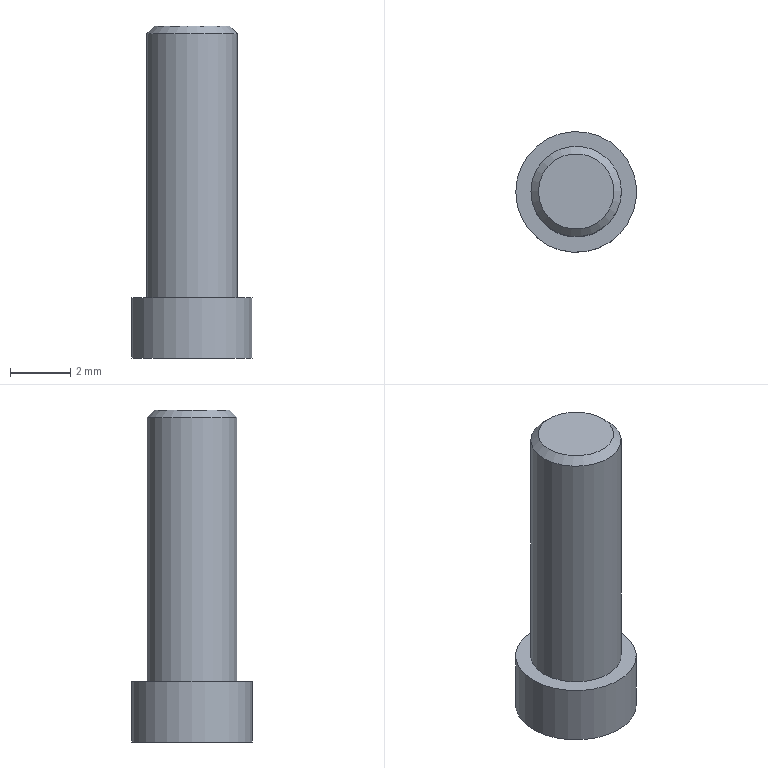Component | NX | SCREW_M3X7_11 | 1 solid | 13 faces | box 4 x 4 x 11 mm | volume 83 mm3 | plane 10 | cylinder 2 | cone 1 | commonest cylinder face diameters 4 x1 3 x1
STEP:
#1=CARTESIAN_POINT('',(0.,0.,0.));
#2=DIRECTION('',(0.,0.,1.));
#3=DIRECTION('',(1.,0.,0.));
#4=AXIS2_PLACEMENT_3D('',#1,#2,#3);
#5=CARTESIAN_POINT('',(12.505,-3.843,-22.));
#6=VERTEX_POINT('',#5);
#7=CARTESIAN_POINT('',(14.505,-3.843,-22.));
#8=DIRECTION('',(0.,0.,-1.));
#9=DIRECTION('',(-1.,0.,0.));
#10=AXIS2_PLACEMENT_3D('',#7,#8,#9);
#11=CIRCLE('',#10,2.);
#12=CARTESIAN_POINT('',(14.505,-3.843,-22.));
#13=DIRECTION('',(0.,0.,-1.));
#14=DIRECTION('',(-1.,0.,0.));
#15=AXIS2_PLACEMENT_3D('',#12,#13,#14);
#16=PLANE('',#15);
#17=CARTESIAN_POINT('',(0.,0.));
#18=DIRECTION('',(1.,0.));
#19=AXIS2_PLACEMENT_2D('',#17,#18);
#20=CIRCLE('',#19,2.);
#21=(GEOMETRIC_REPRESENTATION_CONTEXT(2)PARAMETRIC_REPRESENTATION_CONTEXT()REPRESENTATION_CONTEXT('',''));
#22=DEFINITIONAL_REPRESENTATION('',(#20),#21);
#23=PCURVE('',#16,#22);
#24=CARTESIAN_POINT('',(14.505,-3.843,-22.));
#25=DIRECTION('',(0.,0.,-1.));
#26=DIRECTION('',(-1.,0.,0.));
#27=AXIS2_PLACEMENT_3D('',#24,#25,#26);
#28=CYLINDRICAL_SURFACE('',#27,2.);
#29=CARTESIAN_POINT('',(0.,0.));
#30=DIRECTION('',(1.,0.));
#31=VECTOR('',#30,1.);
#32=LINE('',#29,#31);
#33=(GEOMETRIC_REPRESENTATION_CONTEXT(2)PARAMETRIC_REPRESENTATION_CONTEXT()REPRESENTATION_CONTEXT('',''));
#34=DEFINITIONAL_REPRESENTATION('',(#32),#33);
#35=PCURVE('',#28,#34);
#36=SURFACE_CURVE('',#11,(#23,#35),.PCURVE_S1.);
#37=EDGE_CURVE('',#6,#6,#36,.T.);
#38=ORIENTED_EDGE('',*,*,#37,.F.);
#39=EDGE_LOOP('',(#38));
#40=FACE_BOUND('',#39,.T.);
#41=CARTESIAN_POINT('',(13.005,-3.843,-22.));
#42=VERTEX_POINT('',#41);
#43=CARTESIAN_POINT('',(14.505,-3.843,-22.));
#44=DIRECTION('',(0.,0.,1.));
#45=DIRECTION('',(-1.,0.,0.));
#46=AXIS2_PLACEMENT_3D('',#43,#44,#45);
#47=CIRCLE('',#46,1.5);
#48=CARTESIAN_POINT('',(1.5,0.));
#49=CARTESIAN_POINT('',(1.5,-2.598));
#50=CARTESIAN_POINT('',(-0.75,-1.299));
#51=CARTESIAN_POINT('',(-3.,-0.));
#52=CARTESIAN_POINT('',(-0.75,1.299));
#53=CARTESIAN_POINT('',(1.5,2.598));
#54=CARTESIAN_POINT('',(1.5,0.));
#55=(BOUNDED_CURVE()B_SPLINE_CURVE(2,(#48,#49,#50,#51,#52,#53,#54),.UNSPECIFIED.,.T.,.F.)B_SPLINE_CURVE_WITH_KNOTS((1,2,2,2,2,1),(-2.094,0.,2.094,4.189,6.283,8.378),.UNSPECIFIED.)CURVE()GEOMETRIC_REPRESENTATION_ITEM()RATIONAL_B_SPLINE_CURVE((1.,0.5,1.,0.5,1.,0.5,1.))REPRESENTATION_ITEM(''));
#56=(GEOMETRIC_REPRESENTATION_CONTEXT(2)PARAMETRIC_REPRESENTATION_CONTEXT()REPRESENTATION_CONTEXT('',''));
#57=DEFINITIONAL_REPRESENTATION('',(#55),#56);
#58=PCURVE('',#16,#57);
#59=CARTESIAN_POINT('',(14.505,-3.843,-13.));
#60=DIRECTION('',(0.,0.,-1.));
#61=DIRECTION('',(-1.,0.,0.));
#62=AXIS2_PLACEMENT_3D('',#59,#60,#61);
#63=CYLINDRICAL_SURFACE('',#62,1.5);
#64=CARTESIAN_POINT('',(6.283,9.));
#65=DIRECTION('',(-1.,0.));
#66=VECTOR('',#65,1.);
#67=LINE('',#64,#66);
#68=(GEOMETRIC_REPRESENTATION_CONTEXT(2)PARAMETRIC_REPRESENTATION_CONTEXT()REPRESENTATION_CONTEXT('',''));
#69=DEFINITIONAL_REPRESENTATION('',(#67),#68);
#70=PCURVE('',#63,#69);
#71=SURFACE_CURVE('',#47,(#58,#70),.PCURVE_S1.);
#72=EDGE_CURVE('',#42,#42,#71,.T.);
#73=ORIENTED_EDGE('',*,*,#72,.F.);
#74=EDGE_LOOP('',(#73));
#75=FACE_BOUND('',#74,.T.);
#76=ADVANCED_FACE('',(#40,#75),#16,.F.);
#77=CARTESIAN_POINT('',(12.505,-3.843,-24.));
#78=VERTEX_POINT('',#77);
#79=CARTESIAN_POINT('',(14.505,-3.843,-24.));
#80=DIRECTION('',(0.,0.,-1.));
#81=DIRECTION('',(-1.,0.,0.));
#82=AXIS2_PLACEMENT_3D('',#79,#80,#81);
#83=CIRCLE('',#82,2.);
#84=CARTESIAN_POINT('',(14.505,-3.843,-24.));
#85=DIRECTION('',(0.,0.,-1.));
#86=DIRECTION('',(-1.,0.,0.));
#87=AXIS2_PLACEMENT_3D('',#84,#85,#86);
#88=PLANE('',#87);
#89=CARTESIAN_POINT('',(0.,0.));
#90=DIRECTION('',(1.,0.));
#91=AXIS2_PLACEMENT_2D('',#89,#90);
#92=CIRCLE('',#91,2.);
#93=(GEOMETRIC_REPRESENTATION_CONTEXT(2)PARAMETRIC_REPRESENTATION_CONTEXT()REPRESENTATION_CONTEXT('',''));
#94=DEFINITIONAL_REPRESENTATION('',(#92),#93);
#95=PCURVE('',#88,#94);
#96=CARTESIAN_POINT('',(0.,2.));
#97=DIRECTION('',(1.,0.));
#98=VECTOR('',#97,1.);
#99=LINE('',#96,#98);
#100=(GEOMETRIC_REPRESENTATION_CONTEXT(2)PARAMETRIC_REPRESENTATION_CONTEXT()REPRESENTATION_CONTEXT('',''));
#101=DEFINITIONAL_REPRESENTATION('',(#99),#100);
#102=PCURVE('',#28,#101);
#103=SURFACE_CURVE('',#83,(#95,#102),.PCURVE_S1.);
#104=EDGE_CURVE('',#78,#78,#103,.T.);
#105=ORIENTED_EDGE('',*,*,#104,.T.);
#106=EDGE_LOOP('',(#105));
#107=FACE_BOUND('',#106,.T.);
#108=CARTESIAN_POINT('',(14.505,-5.133,-24.));
#109=VERTEX_POINT('',#108);
#110=CARTESIAN_POINT('',(15.622,-4.488,-24.));
#111=VERTEX_POINT('',#110);
#112=CARTESIAN_POINT('',(14.505,-5.133,-24.));
#113=DIRECTION('',(0.866,0.5,0.));
#114=VECTOR('',#113,1.);
#115=LINE('',#112,#114);
#116=CARTESIAN_POINT('',(-0.,-1.29));
#117=DIRECTION('',(-0.866,0.5));
#118=VECTOR('',#117,1.);
#119=LINE('',#116,#118);
#120=(GEOMETRIC_REPRESENTATION_CONTEXT(2)PARAMETRIC_REPRESENTATION_CONTEXT()REPRESENTATION_CONTEXT('',''));
#121=DEFINITIONAL_REPRESENTATION('',(#119),#120);
#122=PCURVE('',#88,#121);
#123=CARTESIAN_POINT('',(14.505,-5.133,-22.7));
#124=DIRECTION('',(-0.5,0.866,0.));
#125=DIRECTION('',(0.866,0.5,0.));
#126=AXIS2_PLACEMENT_3D('',#123,#124,#125);
#127=PLANE('',#126);
#128=CARTESIAN_POINT('',(0.,1.3));
#129=DIRECTION('',(1.,0.));
#130=VECTOR('',#129,1.);
#131=LINE('',#128,#130);
#132=(GEOMETRIC_REPRESENTATION_CONTEXT(2)PARAMETRIC_REPRESENTATION_CONTEXT()REPRESENTATION_CONTEXT('',''));
#133=DEFINITIONAL_REPRESENTATION('',(#131),#132);
#134=PCURVE('',#127,#133);
#135=SURFACE_CURVE('',#115,(#122,#134),.PCURVE_S1.);
#136=EDGE_CURVE('',#109,#111,#135,.T.);
#137=ORIENTED_EDGE('',*,*,#136,.T.);
#138=CARTESIAN_POINT('',(15.622,-3.198,-24.));
#139=VERTEX_POINT('',#138);
#140=CARTESIAN_POINT('',(15.622,-4.488,-24.));
#141=DIRECTION('',(0.,1.,0.));
#142=VECTOR('',#141,1.);
#143=LINE('',#140,#142);
#144=CARTESIAN_POINT('',(-1.117,-0.645));
#145=DIRECTION('',(0.,1.));
#146=VECTOR('',#145,1.);
#147=LINE('',#144,#146);
#148=(GEOMETRIC_REPRESENTATION_CONTEXT(2)PARAMETRIC_REPRESENTATION_CONTEXT()REPRESENTATION_CONTEXT('',''));
#149=DEFINITIONAL_REPRESENTATION('',(#147),#148);
#150=PCURVE('',#88,#149);
#151=CARTESIAN_POINT('',(15.622,-4.488,-22.7));
#152=DIRECTION('',(-1.,0.,0.));
#153=DIRECTION('',(0.,0.,1.));
#154=AXIS2_PLACEMENT_3D('',#151,#152,#153);
#155=PLANE('',#154);
#156=CARTESIAN_POINT('',(-1.3,0.));
#157=DIRECTION('',(0.,1.));
#158=VECTOR('',#157,1.);
#159=LINE('',#156,#158);
#160=(GEOMETRIC_REPRESENTATION_CONTEXT(2)PARAMETRIC_REPRESENTATION_CONTEXT()REPRESENTATION_CONTEXT('',''));
#161=DEFINITIONAL_REPRESENTATION('',(#159),#160);
#162=PCURVE('',#155,#161);
#163=SURFACE_CURVE('',#143,(#150,#162),.PCURVE_S1.);
#164=EDGE_CURVE('',#111,#139,#163,.T.);
#165=ORIENTED_EDGE('',*,*,#164,.T.);
#166=CARTESIAN_POINT('',(14.505,-2.553,-24.));
#167=VERTEX_POINT('',#166);
#168=CARTESIAN_POINT('',(15.622,-3.198,-24.));
#169=DIRECTION('',(-0.866,0.5,0.));
#170=VECTOR('',#169,1.);
#171=LINE('',#168,#170);
#172=CARTESIAN_POINT('',(-1.117,0.645));
#173=DIRECTION('',(0.866,0.5));
#174=VECTOR('',#173,1.);
#175=LINE('',#172,#174);
#176=(GEOMETRIC_REPRESENTATION_CONTEXT(2)PARAMETRIC_REPRESENTATION_CONTEXT()REPRESENTATION_CONTEXT('',''));
#177=DEFINITIONAL_REPRESENTATION('',(#175),#176);
#178=PCURVE('',#88,#177);
#179=CARTESIAN_POINT('',(15.622,-3.198,-22.7));
#180=DIRECTION('',(-0.5,-0.866,0.));
#181=DIRECTION('',(-0.866,0.5,0.));
#182=AXIS2_PLACEMENT_3D('',#179,#180,#181);
#183=PLANE('',#182);
#184=CARTESIAN_POINT('',(0.,1.3));
#185=DIRECTION('',(1.,0.));
#186=VECTOR('',#185,1.);
#187=LINE('',#184,#186);
#188=(GEOMETRIC_REPRESENTATION_CONTEXT(2)PARAMETRIC_REPRESENTATION_CONTEXT()REPRESENTATION_CONTEXT('',''));
#189=DEFINITIONAL_REPRESENTATION('',(#187),#188);
#190=PCURVE('',#183,#189);
#191=SURFACE_CURVE('',#171,(#178,#190),.PCURVE_S1.);
#192=EDGE_CURVE('',#139,#167,#191,.T.);
#193=ORIENTED_EDGE('',*,*,#192,.T.);
#194=CARTESIAN_POINT('',(13.388,-3.198,-24.));
#195=VERTEX_POINT('',#194);
#196=CARTESIAN_POINT('',(14.505,-2.553,-24.));
#197=DIRECTION('',(-0.866,-0.5,0.));
#198=VECTOR('',#197,1.);
#199=LINE('',#196,#198);
#200=CARTESIAN_POINT('',(0.,1.29));
#201=DIRECTION('',(0.866,-0.5));
#202=VECTOR('',#201,1.);
#203=LINE('',#200,#202);
#204=(GEOMETRIC_REPRESENTATION_CONTEXT(2)PARAMETRIC_REPRESENTATION_CONTEXT()REPRESENTATION_CONTEXT('',''));
#205=DEFINITIONAL_REPRESENTATION('',(#203),#204);
#206=PCURVE('',#88,#205);
#207=CARTESIAN_POINT('',(14.505,-2.553,-22.7));
#208=DIRECTION('',(0.5,-0.866,0.));
#209=DIRECTION('',(-0.866,-0.5,0.));
#210=AXIS2_PLACEMENT_3D('',#207,#208,#209);
#211=PLANE('',#210);
#212=CARTESIAN_POINT('',(0.,1.3));
#213=DIRECTION('',(1.,0.));
#214=VECTOR('',#213,1.);
#215=LINE('',#212,#214);
#216=(GEOMETRIC_REPRESENTATION_CONTEXT(2)PARAMETRIC_REPRESENTATION_CONTEXT()REPRESENTATION_CONTEXT('',''));
#217=DEFINITIONAL_REPRESENTATION('',(#215),#216);
#218=PCURVE('',#211,#217);
#219=SURFACE_CURVE('',#199,(#206,#218),.PCURVE_S1.);
#220=EDGE_CURVE('',#167,#195,#219,.T.);
#221=ORIENTED_EDGE('',*,*,#220,.T.);
#222=CARTESIAN_POINT('',(13.388,-4.488,-24.));
#223=VERTEX_POINT('',#222);
#224=CARTESIAN_POINT('',(13.388,-3.198,-24.));
#225=DIRECTION('',(0.,-1.,0.));
#226=VECTOR('',#225,1.);
#227=LINE('',#224,#226);
#228=CARTESIAN_POINT('',(1.117,0.645));
#229=DIRECTION('',(-0.,-1.));
#230=VECTOR('',#229,1.);
#231=LINE('',#228,#230);
#232=(GEOMETRIC_REPRESENTATION_CONTEXT(2)PARAMETRIC_REPRESENTATION_CONTEXT()REPRESENTATION_CONTEXT('',''));
#233=DEFINITIONAL_REPRESENTATION('',(#231),#232);
#234=PCURVE('',#88,#233);
#235=CARTESIAN_POINT('',(13.388,-3.198,-22.7));
#236=DIRECTION('',(1.,0.,0.));
#237=DIRECTION('',(0.,-1.,0.));
#238=AXIS2_PLACEMENT_3D('',#235,#236,#237);
#239=PLANE('',#238);
#240=CARTESIAN_POINT('',(0.,1.3));
#241=DIRECTION('',(1.,0.));
#242=VECTOR('',#241,1.);
#243=LINE('',#240,#242);
#244=(GEOMETRIC_REPRESENTATION_CONTEXT(2)PARAMETRIC_REPRESENTATION_CONTEXT()REPRESENTATION_CONTEXT('',''));
#245=DEFINITIONAL_REPRESENTATION('',(#243),#244);
#246=PCURVE('',#239,#245);
#247=SURFACE_CURVE('',#227,(#234,#246),.PCURVE_S1.);
#248=EDGE_CURVE('',#195,#223,#247,.T.);
#249=ORIENTED_EDGE('',*,*,#248,.T.);
#250=CARTESIAN_POINT('',(13.388,-4.488,-24.));
#251=DIRECTION('',(0.866,-0.5,0.));
#252=VECTOR('',#251,1.);
#253=LINE('',#250,#252);
#254=CARTESIAN_POINT('',(1.117,-0.645));
#255=DIRECTION('',(-0.866,-0.5));
#256=VECTOR('',#255,1.);
#257=LINE('',#254,#256);
#258=(GEOMETRIC_REPRESENTATION_CONTEXT(2)PARAMETRIC_REPRESENTATION_CONTEXT()REPRESENTATION_CONTEXT('',''));
#259=DEFINITIONAL_REPRESENTATION('',(#257),#258);
#260=PCURVE('',#88,#259);
#261=CARTESIAN_POINT('',(13.388,-4.488,-22.7));
#262=DIRECTION('',(0.5,0.866,0.));
#263=DIRECTION('',(0.866,-0.5,0.));
#264=AXIS2_PLACEMENT_3D('',#261,#262,#263);
#265=PLANE('',#264);
#266=CARTESIAN_POINT('',(0.,1.3));
#267=DIRECTION('',(1.,0.));
#268=VECTOR('',#267,1.);
#269=LINE('',#266,#268);
#270=(GEOMETRIC_REPRESENTATION_CONTEXT(2)PARAMETRIC_REPRESENTATION_CONTEXT()REPRESENTATION_CONTEXT('',''));
#271=DEFINITIONAL_REPRESENTATION('',(#269),#270);
#272=PCURVE('',#265,#271);
#273=SURFACE_CURVE('',#253,(#260,#272),.PCURVE_S1.);
#274=EDGE_CURVE('',#223,#109,#273,.T.);
#275=ORIENTED_EDGE('',*,*,#274,.T.);
#276=EDGE_LOOP('',(#137,#165,#193,#221,#249,#275));
#277=FACE_BOUND('',#276,.T.);
#278=ADVANCED_FACE('',(#107,#277),#88,.T.);
#279=ORIENTED_EDGE('',*,*,#37,.T.);
#280=CARTESIAN_POINT('',(12.505,-3.843,-22.));
#281=CARTESIAN_POINT('',(12.505,-3.843,-24.));
#282=B_SPLINE_CURVE_WITH_KNOTS('',1,(#280,#281),.UNSPECIFIED.,.F.,.F.,(2,2),(0.,2.),.PIECEWISE_BEZIER_KNOTS.);
#283=CARTESIAN_POINT('',(6.283,0.));
#284=DIRECTION('',(0.,1.));
#285=VECTOR('',#284,1.);
#286=LINE('',#283,#285);
#287=(GEOMETRIC_REPRESENTATION_CONTEXT(2)PARAMETRIC_REPRESENTATION_CONTEXT()REPRESENTATION_CONTEXT('',''));
#288=DEFINITIONAL_REPRESENTATION('',(#286),#287);
#289=PCURVE('',#28,#288);
#290=CARTESIAN_POINT('',(0.,0.));
#291=DIRECTION('',(0.,1.));
#292=VECTOR('',#291,1.);
#293=LINE('',#290,#292);
#294=(GEOMETRIC_REPRESENTATION_CONTEXT(2)PARAMETRIC_REPRESENTATION_CONTEXT()REPRESENTATION_CONTEXT('',''));
#295=DEFINITIONAL_REPRESENTATION('',(#293),#294);
#296=PCURVE('',#28,#295);
#297=SEAM_CURVE('',#282,(#289,#296),.PCURVE_S1.);
#298=EDGE_CURVE('',#6,#78,#297,.T.);
#299=ORIENTED_EDGE('',*,*,#298,.T.);
#300=ORIENTED_EDGE('',*,*,#104,.F.);
#301=ORIENTED_EDGE('',*,*,#298,.F.);
#302=EDGE_LOOP('',(#279,#299,#300,#301));
#303=FACE_BOUND('',#302,.T.);
#304=ADVANCED_FACE('',(#303),#28,.T.);
#305=ORIENTED_EDGE('',*,*,#164,.F.);
#306=CARTESIAN_POINT('',(15.622,-4.488,-22.7));
#307=VERTEX_POINT('',#306);
#308=CARTESIAN_POINT('',(15.622,-4.488,-22.7));
#309=DIRECTION('',(0.,0.,-1.));
#310=VECTOR('',#309,1.);
#311=LINE('',#308,#310);
#312=CARTESIAN_POINT('',(0.,0.));
#313=DIRECTION('',(-1.,0.));
#314=VECTOR('',#313,1.);
#315=LINE('',#312,#314);
#316=(GEOMETRIC_REPRESENTATION_CONTEXT(2)PARAMETRIC_REPRESENTATION_CONTEXT()REPRESENTATION_CONTEXT('',''));
#317=DEFINITIONAL_REPRESENTATION('',(#315),#316);
#318=PCURVE('',#155,#317);
#319=CARTESIAN_POINT('',(1.29,0.));
#320=DIRECTION('',(0.,1.));
#321=VECTOR('',#320,1.);
#322=LINE('',#319,#321);
#323=(GEOMETRIC_REPRESENTATION_CONTEXT(2)PARAMETRIC_REPRESENTATION_CONTEXT()REPRESENTATION_CONTEXT('',''));
#324=DEFINITIONAL_REPRESENTATION('',(#322),#323);
#325=PCURVE('',#127,#324);
#326=SURFACE_CURVE('',#311,(#318,#325),.PCURVE_S1.);
#327=EDGE_CURVE('',#307,#111,#326,.T.);
#328=ORIENTED_EDGE('',*,*,#327,.F.);
#329=CARTESIAN_POINT('',(15.622,-3.198,-22.7));
#330=VERTEX_POINT('',#329);
#331=CARTESIAN_POINT('',(15.622,-4.488,-22.7));
#332=DIRECTION('',(0.,1.,0.));
#333=VECTOR('',#332,1.);
#334=LINE('',#331,#333);
#335=CARTESIAN_POINT('',(0.,0.));
#336=DIRECTION('',(0.,1.));
#337=VECTOR('',#336,1.);
#338=LINE('',#335,#337);
#339=(GEOMETRIC_REPRESENTATION_CONTEXT(2)PARAMETRIC_REPRESENTATION_CONTEXT()REPRESENTATION_CONTEXT('',''));
#340=DEFINITIONAL_REPRESENTATION('',(#338),#339);
#341=PCURVE('',#155,#340);
#342=CARTESIAN_POINT('',(15.622,-3.198,-22.7));
#343=DIRECTION('',(0.,0.,1.));
#344=DIRECTION('',(1.,0.,0.));
#345=AXIS2_PLACEMENT_3D('',#342,#343,#344);
#346=PLANE('',#345);
#347=CARTESIAN_POINT('',(0.,-1.29));
#348=DIRECTION('',(0.,1.));
#349=VECTOR('',#348,1.);
#350=LINE('',#347,#349);
#351=(GEOMETRIC_REPRESENTATION_CONTEXT(2)PARAMETRIC_REPRESENTATION_CONTEXT()REPRESENTATION_CONTEXT('',''));
#352=DEFINITIONAL_REPRESENTATION('',(#350),#351);
#353=PCURVE('',#346,#352);
#354=SURFACE_CURVE('',#334,(#341,#353),.PCURVE_S1.);
#355=EDGE_CURVE('',#307,#330,#354,.T.);
#356=ORIENTED_EDGE('',*,*,#355,.T.);
#357=CARTESIAN_POINT('',(15.622,-3.198,-22.7));
#358=DIRECTION('',(0.,0.,-1.));
#359=VECTOR('',#358,1.);
#360=LINE('',#357,#359);
#361=CARTESIAN_POINT('',(0.,1.29));
#362=DIRECTION('',(-1.,0.));
#363=VECTOR('',#362,1.);
#364=LINE('',#361,#363);
#365=(GEOMETRIC_REPRESENTATION_CONTEXT(2)PARAMETRIC_REPRESENTATION_CONTEXT()REPRESENTATION_CONTEXT('',''));
#366=DEFINITIONAL_REPRESENTATION('',(#364),#365);
#367=PCURVE('',#155,#366);
#368=CARTESIAN_POINT('',(0.,0.));
#369=DIRECTION('',(0.,1.));
#370=VECTOR('',#369,1.);
#371=LINE('',#368,#370);
#372=(GEOMETRIC_REPRESENTATION_CONTEXT(2)PARAMETRIC_REPRESENTATION_CONTEXT()REPRESENTATION_CONTEXT('',''));
#373=DEFINITIONAL_REPRESENTATION('',(#371),#372);
#374=PCURVE('',#183,#373);
#375=SURFACE_CURVE('',#360,(#367,#374),.PCURVE_S1.);
#376=EDGE_CURVE('',#330,#139,#375,.T.);
#377=ORIENTED_EDGE('',*,*,#376,.T.);
#378=EDGE_LOOP('',(#305,#328,#356,#377));
#379=FACE_BOUND('',#378,.T.);
#380=ADVANCED_FACE('',(#379),#155,.T.);
#381=ORIENTED_EDGE('',*,*,#192,.F.);
#382=ORIENTED_EDGE('',*,*,#376,.F.);
#383=CARTESIAN_POINT('',(14.505,-2.553,-22.7));
#384=VERTEX_POINT('',#383);
#385=CARTESIAN_POINT('',(15.622,-3.198,-22.7));
#386=DIRECTION('',(-0.866,0.5,0.));
#387=VECTOR('',#386,1.);
#388=LINE('',#385,#387);
#389=CARTESIAN_POINT('',(0.,0.));
#390=DIRECTION('',(1.,0.));
#391=VECTOR('',#390,1.);
#392=LINE('',#389,#391);
#393=(GEOMETRIC_REPRESENTATION_CONTEXT(2)PARAMETRIC_REPRESENTATION_CONTEXT()REPRESENTATION_CONTEXT('',''));
#394=DEFINITIONAL_REPRESENTATION('',(#392),#393);
#395=PCURVE('',#183,#394);
#396=CARTESIAN_POINT('',(0.,0.));
#397=DIRECTION('',(-0.866,0.5));
#398=VECTOR('',#397,1.);
#399=LINE('',#396,#398);
#400=(GEOMETRIC_REPRESENTATION_CONTEXT(2)PARAMETRIC_REPRESENTATION_CONTEXT()REPRESENTATION_CONTEXT('',''));
#401=DEFINITIONAL_REPRESENTATION('',(#399),#400);
#402=PCURVE('',#346,#401);
#403=SURFACE_CURVE('',#388,(#395,#402),.PCURVE_S1.);
#404=EDGE_CURVE('',#330,#384,#403,.T.);
#405=ORIENTED_EDGE('',*,*,#404,.T.);
#406=CARTESIAN_POINT('',(14.505,-2.553,-22.7));
#407=DIRECTION('',(0.,0.,-1.));
#408=VECTOR('',#407,1.);
#409=LINE('',#406,#408);
#410=CARTESIAN_POINT('',(1.29,0.));
#411=DIRECTION('',(0.,1.));
#412=VECTOR('',#411,1.);
#413=LINE('',#410,#412);
#414=(GEOMETRIC_REPRESENTATION_CONTEXT(2)PARAMETRIC_REPRESENTATION_CONTEXT()REPRESENTATION_CONTEXT('',''));
#415=DEFINITIONAL_REPRESENTATION('',(#413),#414);
#416=PCURVE('',#183,#415);
#417=CARTESIAN_POINT('',(-0.,0.));
#418=DIRECTION('',(0.,1.));
#419=VECTOR('',#418,1.);
#420=LINE('',#417,#419);
#421=(GEOMETRIC_REPRESENTATION_CONTEXT(2)PARAMETRIC_REPRESENTATION_CONTEXT()REPRESENTATION_CONTEXT('',''));
#422=DEFINITIONAL_REPRESENTATION('',(#420),#421);
#423=PCURVE('',#211,#422);
#424=SURFACE_CURVE('',#409,(#416,#423),.PCURVE_S1.);
#425=EDGE_CURVE('',#384,#167,#424,.T.);
#426=ORIENTED_EDGE('',*,*,#425,.T.);
#427=EDGE_LOOP('',(#381,#382,#405,#426));
#428=FACE_BOUND('',#427,.T.);
#429=ADVANCED_FACE('',(#428),#183,.T.);
#430=ORIENTED_EDGE('',*,*,#220,.F.);
#431=ORIENTED_EDGE('',*,*,#425,.F.);
#432=CARTESIAN_POINT('',(13.388,-3.198,-22.7));
#433=VERTEX_POINT('',#432);
#434=CARTESIAN_POINT('',(14.505,-2.553,-22.7));
#435=DIRECTION('',(-0.866,-0.5,0.));
#436=VECTOR('',#435,1.);
#437=LINE('',#434,#436);
#438=CARTESIAN_POINT('',(0.,0.));
#439=DIRECTION('',(1.,0.));
#440=VECTOR('',#439,1.);
#441=LINE('',#438,#440);
#442=(GEOMETRIC_REPRESENTATION_CONTEXT(2)PARAMETRIC_REPRESENTATION_CONTEXT()REPRESENTATION_CONTEXT('',''));
#443=DEFINITIONAL_REPRESENTATION('',(#441),#442);
#444=PCURVE('',#211,#443);
#445=CARTESIAN_POINT('',(-1.117,0.645));
#446=DIRECTION('',(-0.866,-0.5));
#447=VECTOR('',#446,1.);
#448=LINE('',#445,#447);
#449=(GEOMETRIC_REPRESENTATION_CONTEXT(2)PARAMETRIC_REPRESENTATION_CONTEXT()REPRESENTATION_CONTEXT('',''));
#450=DEFINITIONAL_REPRESENTATION('',(#448),#449);
#451=PCURVE('',#346,#450);
#452=SURFACE_CURVE('',#437,(#444,#451),.PCURVE_S1.);
#453=EDGE_CURVE('',#384,#433,#452,.T.);
#454=ORIENTED_EDGE('',*,*,#453,.T.);
#455=CARTESIAN_POINT('',(13.388,-3.198,-22.7));
#456=DIRECTION('',(0.,0.,-1.));
#457=VECTOR('',#456,1.);
#458=LINE('',#455,#457);
#459=CARTESIAN_POINT('',(1.29,0.));
#460=DIRECTION('',(0.,1.));
#461=VECTOR('',#460,1.);
#462=LINE('',#459,#461);
#463=(GEOMETRIC_REPRESENTATION_CONTEXT(2)PARAMETRIC_REPRESENTATION_CONTEXT()REPRESENTATION_CONTEXT('',''));
#464=DEFINITIONAL_REPRESENTATION('',(#462),#463);
#465=PCURVE('',#211,#464);
#466=CARTESIAN_POINT('',(0.,0.));
#467=DIRECTION('',(0.,1.));
#468=VECTOR('',#467,1.);
#469=LINE('',#466,#468);
#470=(GEOMETRIC_REPRESENTATION_CONTEXT(2)PARAMETRIC_REPRESENTATION_CONTEXT()REPRESENTATION_CONTEXT('',''));
#471=DEFINITIONAL_REPRESENTATION('',(#469),#470);
#472=PCURVE('',#239,#471);
#473=SURFACE_CURVE('',#458,(#465,#472),.PCURVE_S1.);
#474=EDGE_CURVE('',#433,#195,#473,.T.);
#475=ORIENTED_EDGE('',*,*,#474,.T.);
#476=EDGE_LOOP('',(#430,#431,#454,#475));
#477=FACE_BOUND('',#476,.T.);
#478=ADVANCED_FACE('',(#477),#211,.T.);
#479=ORIENTED_EDGE('',*,*,#248,.F.);
#480=ORIENTED_EDGE('',*,*,#474,.F.);
#481=CARTESIAN_POINT('',(13.388,-4.488,-22.7));
#482=VERTEX_POINT('',#481);
#483=CARTESIAN_POINT('',(13.388,-3.198,-22.7));
#484=DIRECTION('',(0.,-1.,0.));
#485=VECTOR('',#484,1.);
#486=LINE('',#483,#485);
#487=CARTESIAN_POINT('',(0.,0.));
#488=DIRECTION('',(1.,0.));
#489=VECTOR('',#488,1.);
#490=LINE('',#487,#489);
#491=(GEOMETRIC_REPRESENTATION_CONTEXT(2)PARAMETRIC_REPRESENTATION_CONTEXT()REPRESENTATION_CONTEXT('',''));
#492=DEFINITIONAL_REPRESENTATION('',(#490),#491);
#493=PCURVE('',#239,#492);
#494=CARTESIAN_POINT('',(-2.234,-0.));
#495=DIRECTION('',(0.,-1.));
#496=VECTOR('',#495,1.);
#497=LINE('',#494,#496);
#498=(GEOMETRIC_REPRESENTATION_CONTEXT(2)PARAMETRIC_REPRESENTATION_CONTEXT()REPRESENTATION_CONTEXT('',''));
#499=DEFINITIONAL_REPRESENTATION('',(#497),#498);
#500=PCURVE('',#346,#499);
#501=SURFACE_CURVE('',#486,(#493,#500),.PCURVE_S1.);
#502=EDGE_CURVE('',#433,#482,#501,.T.);
#503=ORIENTED_EDGE('',*,*,#502,.T.);
#504=CARTESIAN_POINT('',(13.388,-4.488,-22.7));
#505=DIRECTION('',(0.,0.,-1.));
#506=VECTOR('',#505,1.);
#507=LINE('',#504,#506);
#508=CARTESIAN_POINT('',(1.29,0.));
#509=DIRECTION('',(0.,1.));
#510=VECTOR('',#509,1.);
#511=LINE('',#508,#510);
#512=(GEOMETRIC_REPRESENTATION_CONTEXT(2)PARAMETRIC_REPRESENTATION_CONTEXT()REPRESENTATION_CONTEXT('',''));
#513=DEFINITIONAL_REPRESENTATION('',(#511),#512);
#514=PCURVE('',#239,#513);
#515=CARTESIAN_POINT('',(0.,0.));
#516=DIRECTION('',(0.,1.));
#517=VECTOR('',#516,1.);
#518=LINE('',#515,#517);
#519=(GEOMETRIC_REPRESENTATION_CONTEXT(2)PARAMETRIC_REPRESENTATION_CONTEXT()REPRESENTATION_CONTEXT('',''));
#520=DEFINITIONAL_REPRESENTATION('',(#518),#519);
#521=PCURVE('',#265,#520);
#522=SURFACE_CURVE('',#507,(#514,#521),.PCURVE_S1.);
#523=EDGE_CURVE('',#482,#223,#522,.T.);
#524=ORIENTED_EDGE('',*,*,#523,.T.);
#525=EDGE_LOOP('',(#479,#480,#503,#524));
#526=FACE_BOUND('',#525,.T.);
#527=ADVANCED_FACE('',(#526),#239,.T.);
#528=ORIENTED_EDGE('',*,*,#274,.F.);
#529=ORIENTED_EDGE('',*,*,#523,.F.);
#530=CARTESIAN_POINT('',(14.505,-5.133,-22.7));
#531=VERTEX_POINT('',#530);
#532=CARTESIAN_POINT('',(13.388,-4.488,-22.7));
#533=DIRECTION('',(0.866,-0.5,0.));
#534=VECTOR('',#533,1.);
#535=LINE('',#532,#534);
#536=CARTESIAN_POINT('',(0.,0.));
#537=DIRECTION('',(1.,0.));
#538=VECTOR('',#537,1.);
#539=LINE('',#536,#538);
#540=(GEOMETRIC_REPRESENTATION_CONTEXT(2)PARAMETRIC_REPRESENTATION_CONTEXT()REPRESENTATION_CONTEXT('',''));
#541=DEFINITIONAL_REPRESENTATION('',(#539),#540);
#542=PCURVE('',#265,#541);
#543=CARTESIAN_POINT('',(-2.234,-1.29));
#544=DIRECTION('',(0.866,-0.5));
#545=VECTOR('',#544,1.);
#546=LINE('',#543,#545);
#547=(GEOMETRIC_REPRESENTATION_CONTEXT(2)PARAMETRIC_REPRESENTATION_CONTEXT()REPRESENTATION_CONTEXT('',''));
#548=DEFINITIONAL_REPRESENTATION('',(#546),#547);
#549=PCURVE('',#346,#548);
#550=SURFACE_CURVE('',#535,(#542,#549),.PCURVE_S1.);
#551=EDGE_CURVE('',#482,#531,#550,.T.);
#552=ORIENTED_EDGE('',*,*,#551,.T.);
#553=CARTESIAN_POINT('',(14.505,-5.133,-22.7));
#554=DIRECTION('',(0.,0.,-1.));
#555=VECTOR('',#554,1.);
#556=LINE('',#553,#555);
#557=CARTESIAN_POINT('',(1.29,0.));
#558=DIRECTION('',(0.,1.));
#559=VECTOR('',#558,1.);
#560=LINE('',#557,#559);
#561=(GEOMETRIC_REPRESENTATION_CONTEXT(2)PARAMETRIC_REPRESENTATION_CONTEXT()REPRESENTATION_CONTEXT('',''));
#562=DEFINITIONAL_REPRESENTATION('',(#560),#561);
#563=PCURVE('',#265,#562);
#564=CARTESIAN_POINT('',(-0.,0.));
#565=DIRECTION('',(0.,1.));
#566=VECTOR('',#565,1.);
#567=LINE('',#564,#566);
#568=(GEOMETRIC_REPRESENTATION_CONTEXT(2)PARAMETRIC_REPRESENTATION_CONTEXT()REPRESENTATION_CONTEXT('',''));
#569=DEFINITIONAL_REPRESENTATION('',(#567),#568);
#570=PCURVE('',#127,#569);
#571=SURFACE_CURVE('',#556,(#563,#570),.PCURVE_S1.);
#572=EDGE_CURVE('',#531,#109,#571,.T.);
#573=ORIENTED_EDGE('',*,*,#572,.T.);
#574=EDGE_LOOP('',(#528,#529,#552,#573));
#575=FACE_BOUND('',#574,.T.);
#576=ADVANCED_FACE('',(#575),#265,.T.);
#577=ORIENTED_EDGE('',*,*,#136,.F.);
#578=ORIENTED_EDGE('',*,*,#572,.F.);
#579=CARTESIAN_POINT('',(14.505,-5.133,-22.7));
#580=DIRECTION('',(0.866,0.5,0.));
#581=VECTOR('',#580,1.);
#582=LINE('',#579,#581);
#583=CARTESIAN_POINT('',(0.,0.));
#584=DIRECTION('',(1.,0.));
#585=VECTOR('',#584,1.);
#586=LINE('',#583,#585);
#587=(GEOMETRIC_REPRESENTATION_CONTEXT(2)PARAMETRIC_REPRESENTATION_CONTEXT()REPRESENTATION_CONTEXT('',''));
#588=DEFINITIONAL_REPRESENTATION('',(#586),#587);
#589=PCURVE('',#127,#588);
#590=CARTESIAN_POINT('',(-1.117,-1.935));
#591=DIRECTION('',(0.866,0.5));
#592=VECTOR('',#591,1.);
#593=LINE('',#590,#592);
#594=(GEOMETRIC_REPRESENTATION_CONTEXT(2)PARAMETRIC_REPRESENTATION_CONTEXT()REPRESENTATION_CONTEXT('',''));
#595=DEFINITIONAL_REPRESENTATION('',(#593),#594);
#596=PCURVE('',#346,#595);
#597=SURFACE_CURVE('',#582,(#589,#596),.PCURVE_S1.);
#598=EDGE_CURVE('',#531,#307,#597,.T.);
#599=ORIENTED_EDGE('',*,*,#598,.T.);
#600=ORIENTED_EDGE('',*,*,#327,.T.);
#601=EDGE_LOOP('',(#577,#578,#599,#600));
#602=FACE_BOUND('',#601,.T.);
#603=ADVANCED_FACE('',(#602),#127,.T.);
#604=ORIENTED_EDGE('',*,*,#355,.F.);
#605=ORIENTED_EDGE('',*,*,#598,.F.);
#606=ORIENTED_EDGE('',*,*,#551,.F.);
#607=ORIENTED_EDGE('',*,*,#502,.F.);
#608=ORIENTED_EDGE('',*,*,#453,.F.);
#609=ORIENTED_EDGE('',*,*,#404,.F.);
#610=EDGE_LOOP('',(#604,#605,#606,#607,#608,#609));
#611=FACE_BOUND('',#610,.T.);
#612=ADVANCED_FACE('',(#611),#346,.F.);
#613=CARTESIAN_POINT('',(16.005,-3.843,-13.25));
#614=VERTEX_POINT('',#613);
#615=CARTESIAN_POINT('',(13.005,-3.843,-13.25));
#616=VERTEX_POINT('',#615);
#617=CARTESIAN_POINT('',(14.505,-3.843,-13.25));
#618=DIRECTION('',(0.,0.,-1.));
#619=DIRECTION('',(1.,0.,0.));
#620=AXIS2_PLACEMENT_3D('',#617,#618,#619);
#621=CIRCLE('',#620,1.5);
#622=CARTESIAN_POINT('',(3.142,0.25));
#623=DIRECTION('',(1.,0.));
#624=VECTOR('',#623,1.);
#625=LINE('',#622,#624);
#626=(GEOMETRIC_REPRESENTATION_CONTEXT(2)PARAMETRIC_REPRESENTATION_CONTEXT()REPRESENTATION_CONTEXT('',''));
#627=DEFINITIONAL_REPRESENTATION('',(#625),#626);
#628=PCURVE('',#63,#627);
#629=CARTESIAN_POINT('',(14.505,-3.843,-13.));
#630=DIRECTION('',(0.,0.,-1.));
#631=DIRECTION('',(-1.,0.,0.));
#632=AXIS2_PLACEMENT_3D('',#629,#630,#631);
#633=CONICAL_SURFACE('',#632,1.25,0.7854);
#634=CARTESIAN_POINT('',(3.142,0.25));
#635=DIRECTION('',(1.,0.));
#636=VECTOR('',#635,1.);
#637=LINE('',#634,#636);
#638=(GEOMETRIC_REPRESENTATION_CONTEXT(2)PARAMETRIC_REPRESENTATION_CONTEXT()REPRESENTATION_CONTEXT('',''));
#639=DEFINITIONAL_REPRESENTATION('',(#637),#638);
#640=PCURVE('',#633,#639);
#641=SURFACE_CURVE('',#621,(#628,#640),.PCURVE_S1.);
#642=EDGE_CURVE('',#614,#616,#641,.T.);
#643=ORIENTED_EDGE('',*,*,#642,.T.);
#644=CARTESIAN_POINT('',(13.005,-3.843,-13.25));
#645=CARTESIAN_POINT('',(13.005,-3.843,-22.));
#646=B_SPLINE_CURVE_WITH_KNOTS('',1,(#644,#645),.UNSPECIFIED.,.F.,.F.,(2,2),(0.25,9.),.PIECEWISE_BEZIER_KNOTS.);
#647=CARTESIAN_POINT('',(6.283,0.));
#648=DIRECTION('',(0.,1.));
#649=VECTOR('',#648,1.);
#650=LINE('',#647,#649);
#651=(GEOMETRIC_REPRESENTATION_CONTEXT(2)PARAMETRIC_REPRESENTATION_CONTEXT()REPRESENTATION_CONTEXT('',''));
#652=DEFINITIONAL_REPRESENTATION('',(#650),#651);
#653=PCURVE('',#63,#652);
#654=CARTESIAN_POINT('',(0.,0.));
#655=DIRECTION('',(0.,1.));
#656=VECTOR('',#655,1.);
#657=LINE('',#654,#656);
#658=(GEOMETRIC_REPRESENTATION_CONTEXT(2)PARAMETRIC_REPRESENTATION_CONTEXT()REPRESENTATION_CONTEXT('',''));
#659=DEFINITIONAL_REPRESENTATION('',(#657),#658);
#660=PCURVE('',#63,#659);
#661=SEAM_CURVE('',#646,(#653,#660),.PCURVE_S1.);
#662=EDGE_CURVE('',#616,#42,#661,.T.);
#663=ORIENTED_EDGE('',*,*,#662,.T.);
#664=ORIENTED_EDGE('',*,*,#72,.T.);
#665=ORIENTED_EDGE('',*,*,#662,.F.);
#666=CARTESIAN_POINT('',(14.505,-3.843,-13.25));
#667=DIRECTION('',(0.,0.,-1.));
#668=DIRECTION('',(1.,0.,0.));
#669=AXIS2_PLACEMENT_3D('',#666,#667,#668);
#670=CIRCLE('',#669,1.5);
#671=CARTESIAN_POINT('',(-3.142,0.25));
#672=DIRECTION('',(1.,0.));
#673=VECTOR('',#672,1.);
#674=LINE('',#671,#673);
#675=(GEOMETRIC_REPRESENTATION_CONTEXT(2)PARAMETRIC_REPRESENTATION_CONTEXT()REPRESENTATION_CONTEXT('',''));
#676=DEFINITIONAL_REPRESENTATION('',(#674),#675);
#677=PCURVE('',#63,#676);
#678=CARTESIAN_POINT('',(3.142,0.25));
#679=DIRECTION('',(1.,0.));
#680=VECTOR('',#679,1.);
#681=LINE('',#678,#680);
#682=(GEOMETRIC_REPRESENTATION_CONTEXT(2)PARAMETRIC_REPRESENTATION_CONTEXT()REPRESENTATION_CONTEXT('',''));
#683=DEFINITIONAL_REPRESENTATION('',(#681),#682);
#684=PCURVE('',#633,#683);
#685=SURFACE_CURVE('',#670,(#677,#684),.PCURVE_S1.);
#686=EDGE_CURVE('',#616,#614,#685,.T.);
#687=ORIENTED_EDGE('',*,*,#686,.T.);
#688=EDGE_LOOP('',(#643,#663,#664,#665,#687));
#689=FACE_BOUND('',#688,.T.);
#690=ADVANCED_FACE('',(#689),#63,.T.);
#691=CARTESIAN_POINT('',(15.755,-3.843,-13.));
#692=VERTEX_POINT('',#691);
#693=CARTESIAN_POINT('',(14.505,-3.843,-13.));
#694=DIRECTION('',(0.,0.,1.));
#695=DIRECTION('',(1.,0.,0.));
#696=AXIS2_PLACEMENT_3D('',#693,#694,#695);
#697=CIRCLE('',#696,1.25);
#698=CARTESIAN_POINT('',(14.505,-3.843,-13.));
#699=DIRECTION('',(0.,0.,1.));
#700=DIRECTION('',(1.,0.,0.));
#701=AXIS2_PLACEMENT_3D('',#698,#699,#700);
#702=PLANE('',#701);
#703=CARTESIAN_POINT('',(0.,0.));
#704=DIRECTION('',(1.,0.));
#705=AXIS2_PLACEMENT_2D('',#703,#704);
#706=CIRCLE('',#705,1.25);
#707=(GEOMETRIC_REPRESENTATION_CONTEXT(2)PARAMETRIC_REPRESENTATION_CONTEXT()REPRESENTATION_CONTEXT('',''));
#708=DEFINITIONAL_REPRESENTATION('',(#706),#707);
#709=PCURVE('',#702,#708);
#710=CARTESIAN_POINT('',(9.425,0.));
#711=DIRECTION('',(-1.,0.));
#712=VECTOR('',#711,1.);
#713=LINE('',#710,#712);
#714=(GEOMETRIC_REPRESENTATION_CONTEXT(2)PARAMETRIC_REPRESENTATION_CONTEXT()REPRESENTATION_CONTEXT('',''));
#715=DEFINITIONAL_REPRESENTATION('',(#713),#714);
#716=PCURVE('',#633,#715);
#717=SURFACE_CURVE('',#697,(#709,#716),.PCURVE_S1.);
#718=EDGE_CURVE('',#692,#692,#717,.T.);
#719=ORIENTED_EDGE('',*,*,#718,.T.);
#720=EDGE_LOOP('',(#719));
#721=FACE_BOUND('',#720,.T.);
#722=ADVANCED_FACE('',(#721),#702,.T.);
#723=ORIENTED_EDGE('',*,*,#642,.F.);
#724=CARTESIAN_POINT('',(15.755,-3.843,-13.));
#725=CARTESIAN_POINT('',(16.005,-3.843,-13.25));
#726=B_SPLINE_CURVE_WITH_KNOTS('',1,(#724,#725),.UNSPECIFIED.,.F.,.F.,(2,2),(0.,0.3536),.PIECEWISE_BEZIER_KNOTS.);
#727=CARTESIAN_POINT('',(3.142,0.));
#728=DIRECTION('',(0.,1.));
#729=VECTOR('',#728,1.);
#730=LINE('',#727,#729);
#731=(GEOMETRIC_REPRESENTATION_CONTEXT(2)PARAMETRIC_REPRESENTATION_CONTEXT()REPRESENTATION_CONTEXT('',''));
#732=DEFINITIONAL_REPRESENTATION('',(#730),#731);
#733=PCURVE('',#633,#732);
#734=CARTESIAN_POINT('',(9.425,0.));
#735=DIRECTION('',(0.,1.));
#736=VECTOR('',#735,1.);
#737=LINE('',#734,#736);
#738=(GEOMETRIC_REPRESENTATION_CONTEXT(2)PARAMETRIC_REPRESENTATION_CONTEXT()REPRESENTATION_CONTEXT('',''));
#739=DEFINITIONAL_REPRESENTATION('',(#737),#738);
#740=PCURVE('',#633,#739);
#741=SEAM_CURVE('',#726,(#733,#740),.PCURVE_S1.);
#742=EDGE_CURVE('',#692,#614,#741,.T.);
#743=ORIENTED_EDGE('',*,*,#742,.F.);
#744=ORIENTED_EDGE('',*,*,#718,.F.);
#745=ORIENTED_EDGE('',*,*,#742,.T.);
#746=ORIENTED_EDGE('',*,*,#686,.F.);
#747=EDGE_LOOP('',(#723,#743,#744,#745,#746));
#748=FACE_BOUND('',#747,.T.);
#749=ADVANCED_FACE('',(#748),#633,.T.);
#750=CLOSED_SHELL('',(#76,#278,#304,#380,#429,#478,#527,#576,#603,#612,#690,#722,#749));
#751=MANIFOLD_SOLID_BREP('',#750);
#752=(LENGTH_UNIT()NAMED_UNIT(*)SI_UNIT(.MILLI.,.METRE.));
#753=UNCERTAINTY_MEASURE_WITH_UNIT(LENGTH_MEASURE(0.000002),#752,'','');
#754=(NAMED_UNIT(*)PLANE_ANGLE_UNIT()SI_UNIT($,.RADIAN.));
#755=(NAMED_UNIT(*)SI_UNIT($,.STERADIAN.)SOLID_ANGLE_UNIT());
#756=(GEOMETRIC_REPRESENTATION_CONTEXT(3)GLOBAL_UNCERTAINTY_ASSIGNED_CONTEXT((#753))GLOBAL_UNIT_ASSIGNED_CONTEXT((#752,#754,#755))REPRESENTATION_CONTEXT('',''));
#757=ADVANCED_BREP_SHAPE_REPRESENTATION('',(#4,#751),#756);